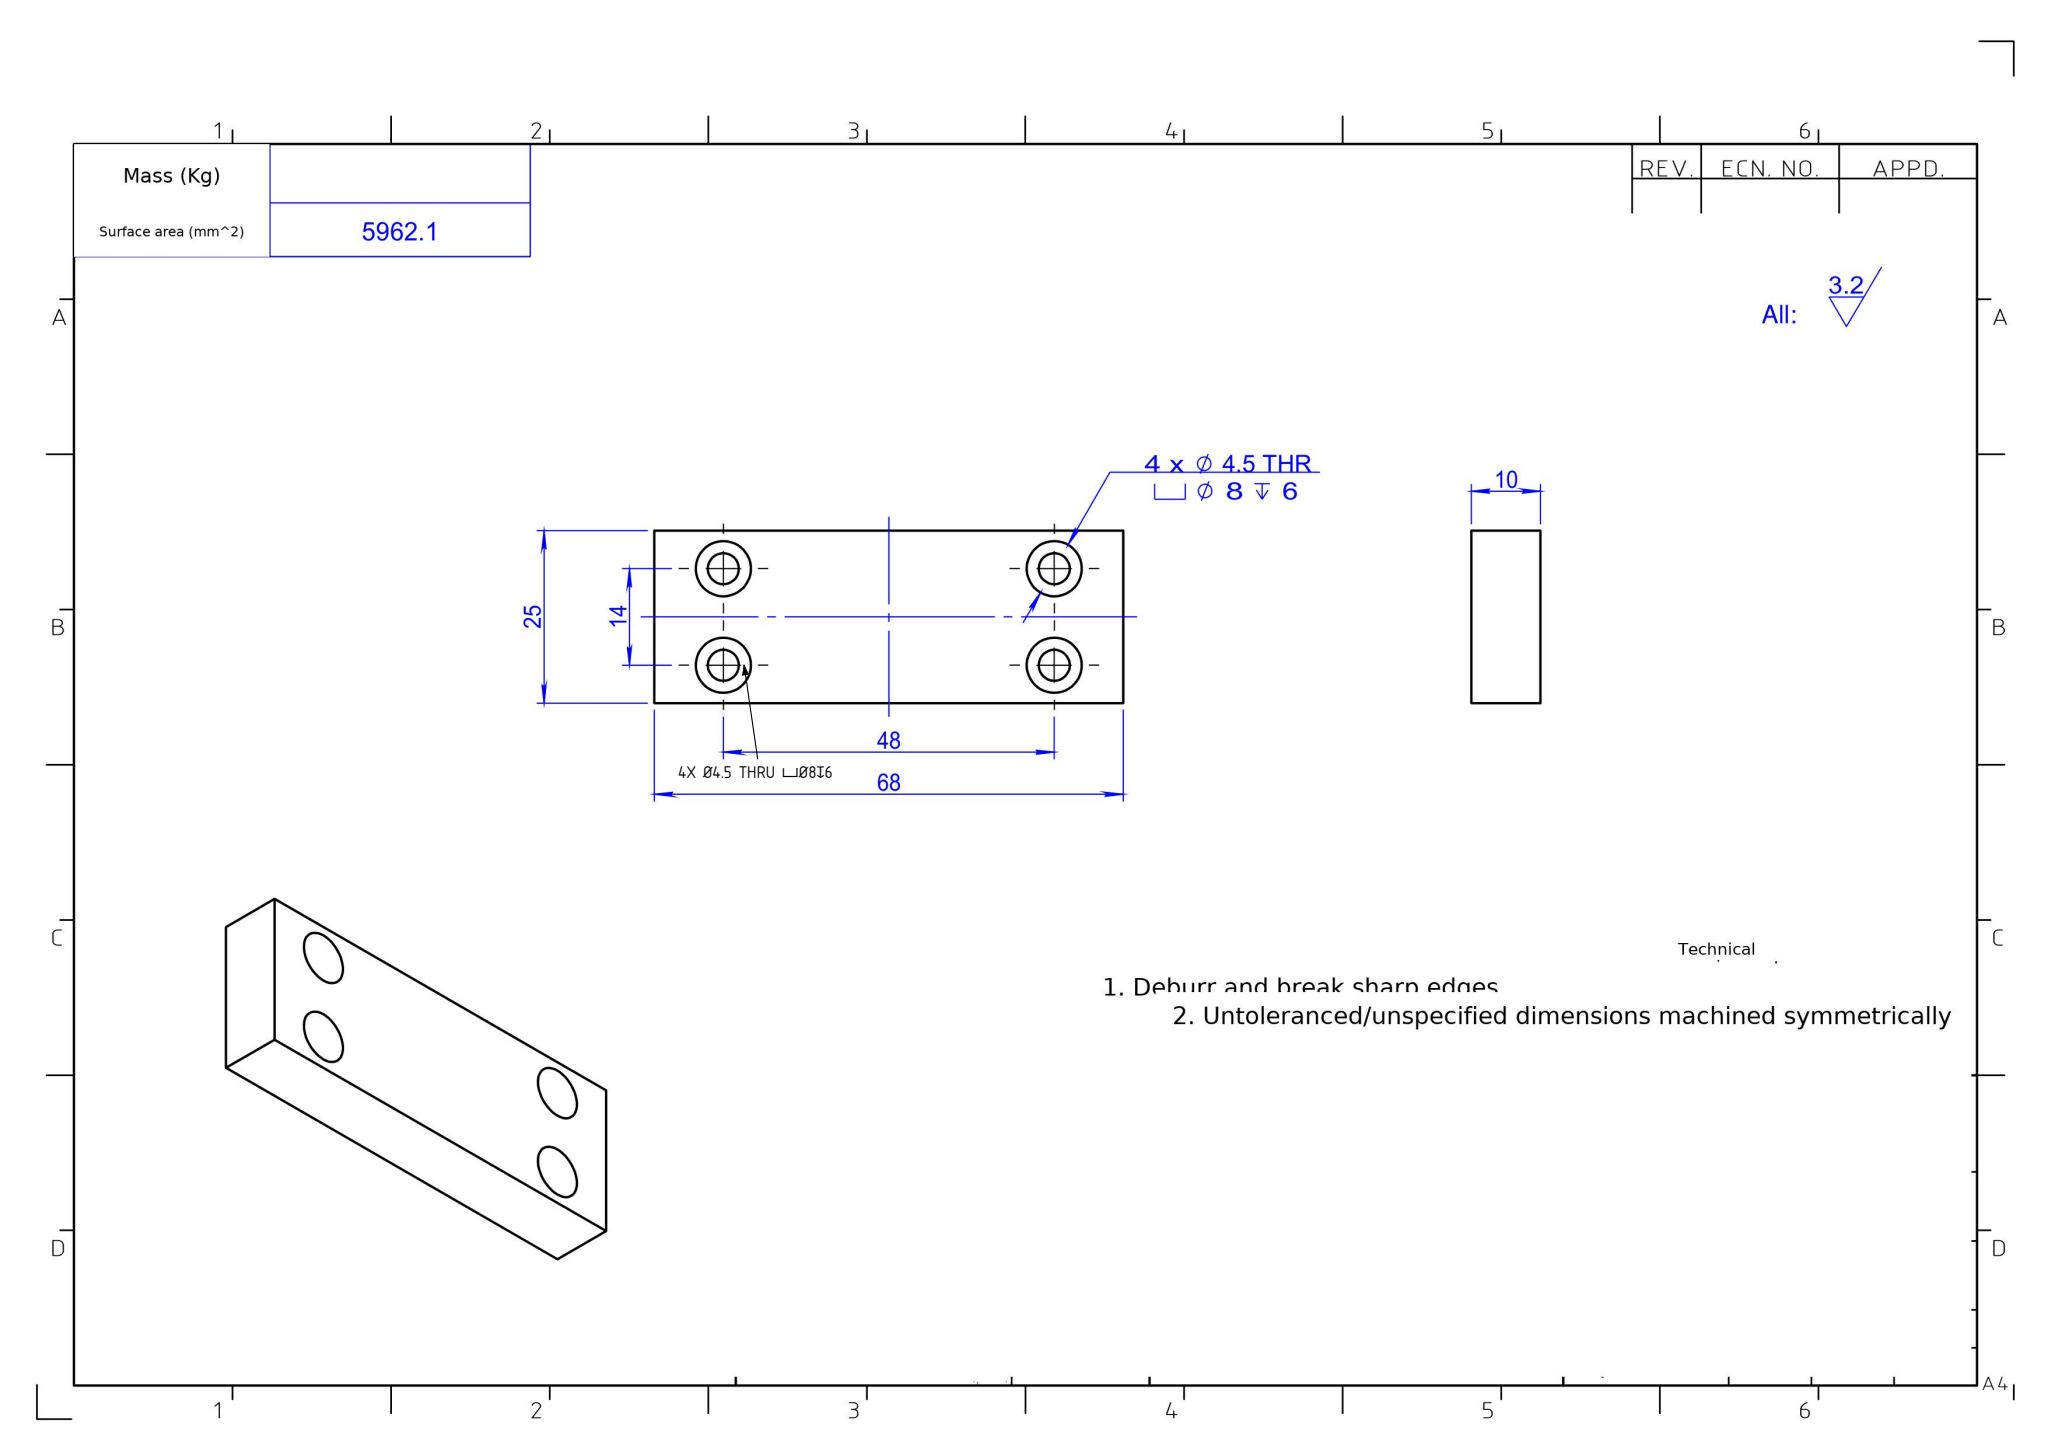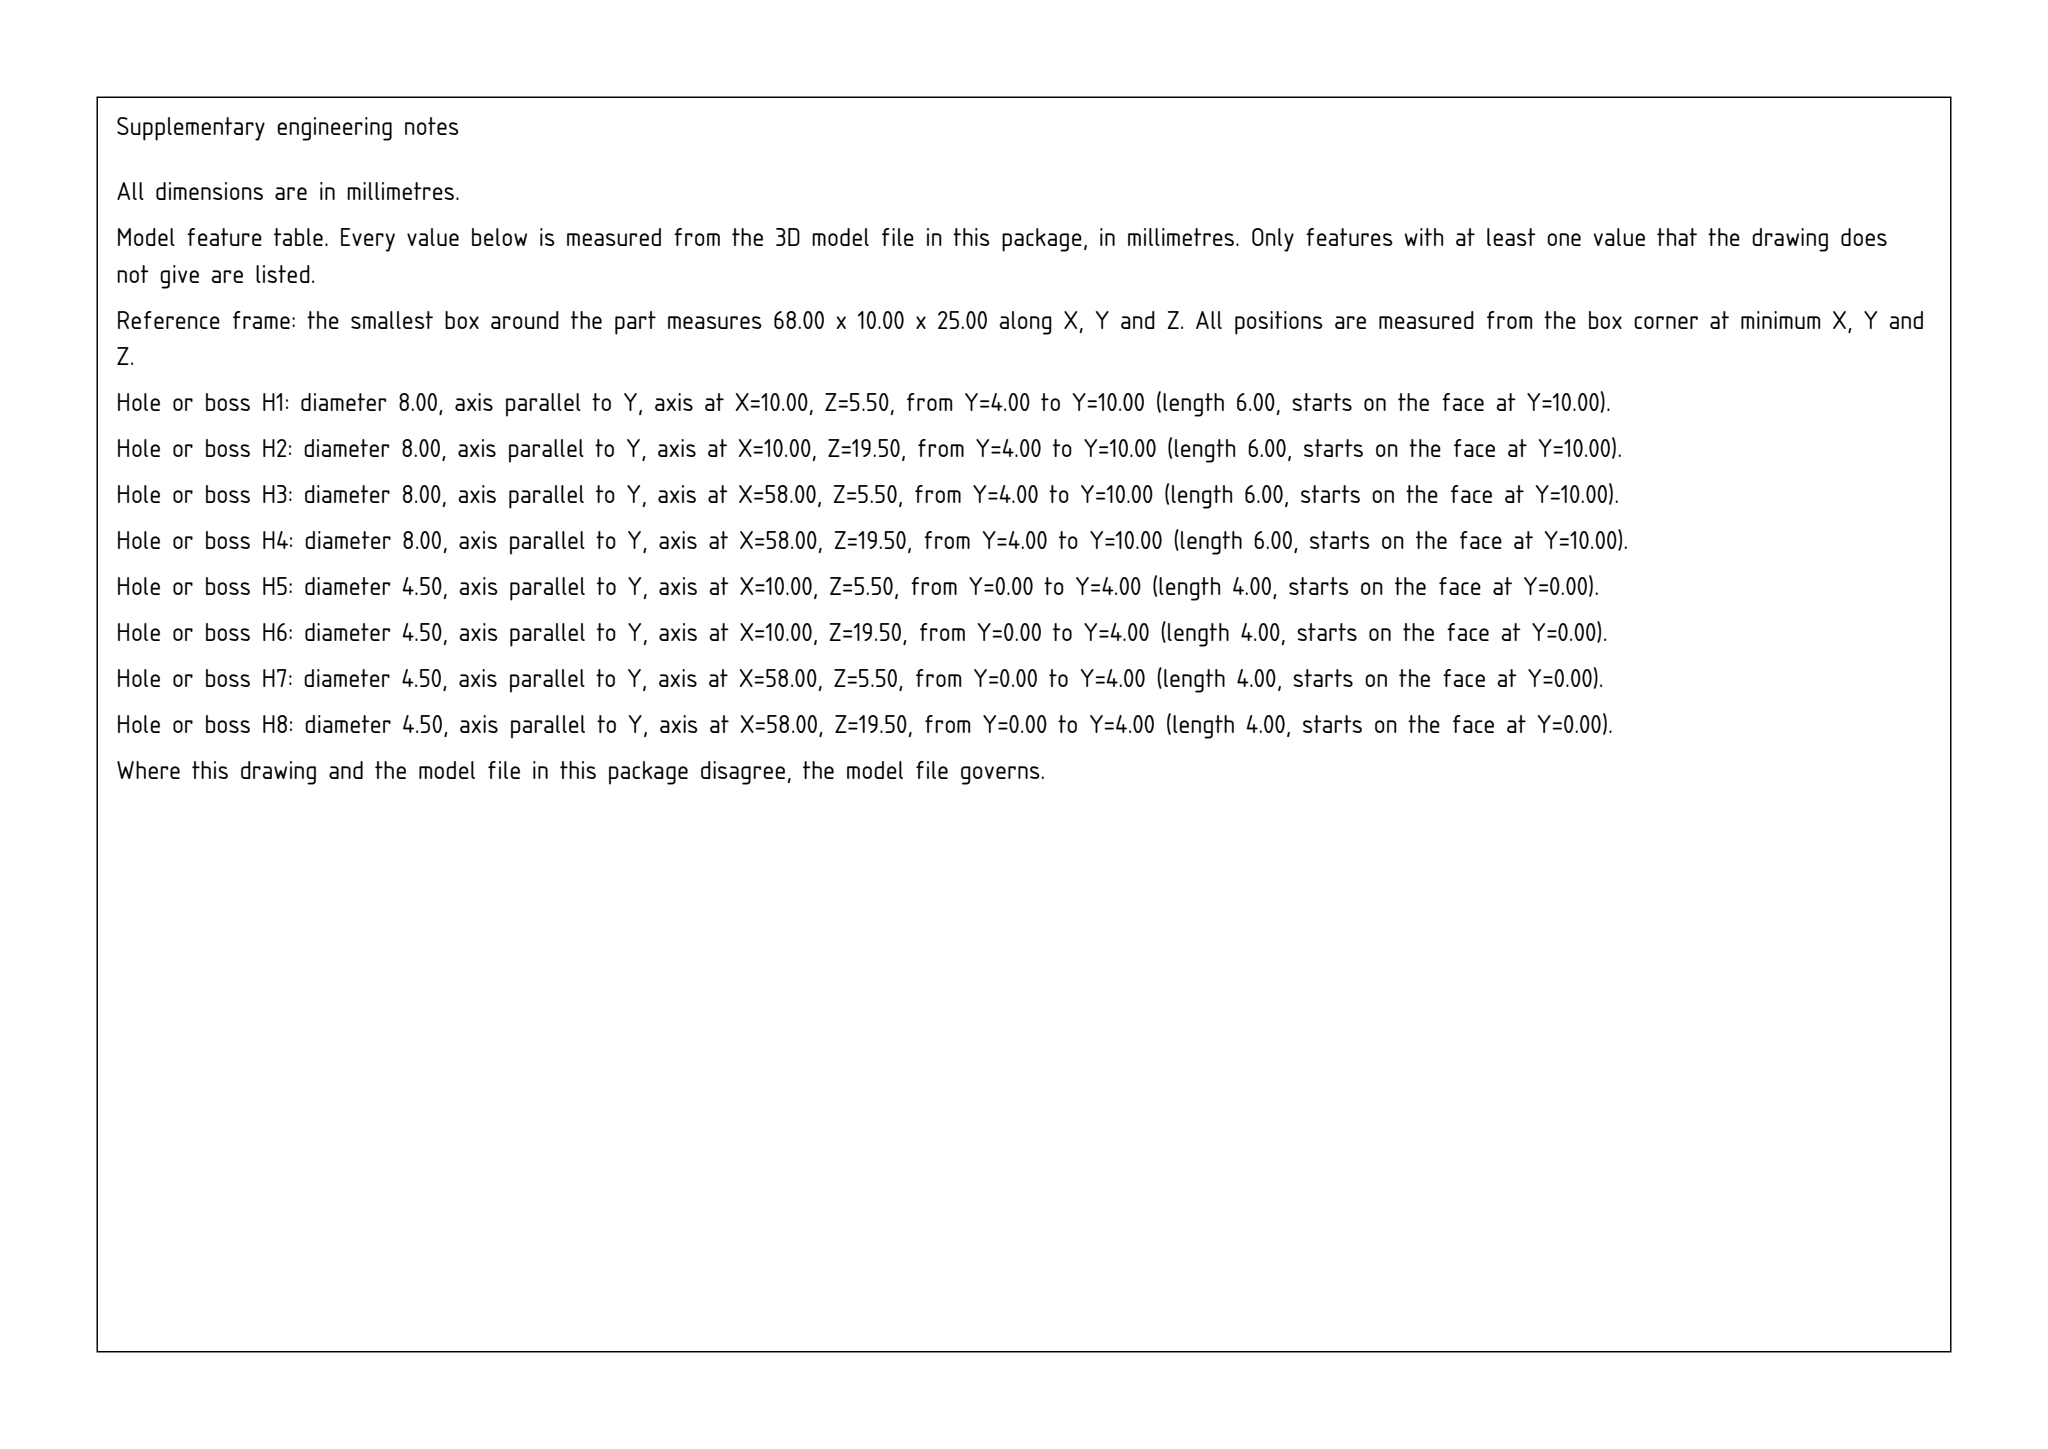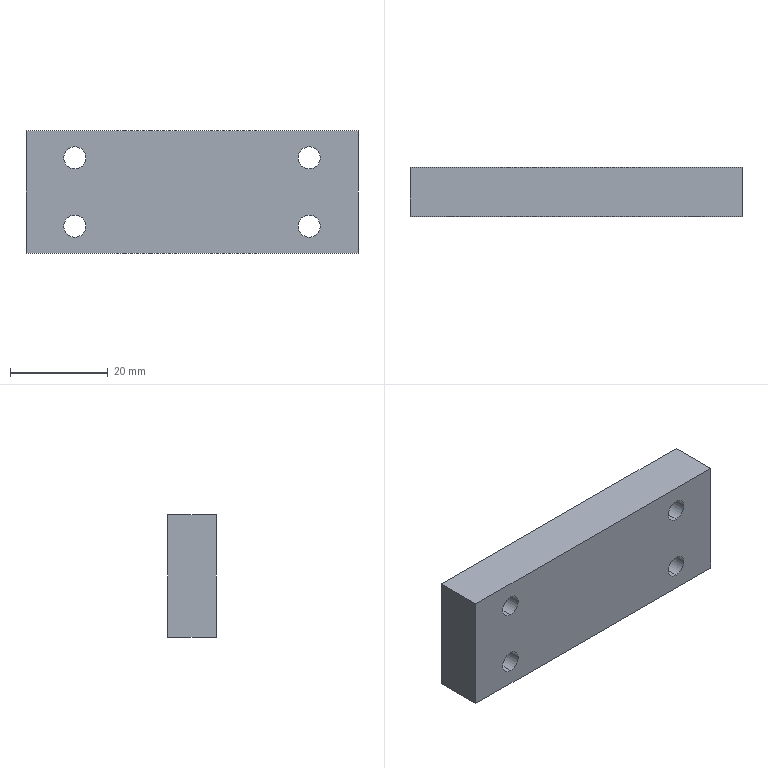Part | SolidWorks | mm | 1 solid | 26 faces | box 68 x 10 x 25 mm | volume 15539 mm3 | cylinder 16 | plane 10 | commonest cylinder face diameters 4.5 x8 8 x8
Drawing notes:
4X Ø4.5 THRU, C'BORE Ø8 DP 6 FROM OPP FACE | from the solid: Ø4.5 bores y=0->4 (4 deep) and Ø8 bores y=4->10 (6 deep) in 10 thk plate; 4+6=10 = full thickness, so Ø4.5 breaks through
build123d program:
from build123d import *

# Parameters (mm, degrees)
SKETCH1_W                                            = 68
SKETCH1_H                                            = 25
EXTRUDE1_DEPTH                                       = 10
COUNTERBORE_FOR_M4_HEX_SOCKET_HEAD_CAP_S_D           = 4.5
COUNTERBORE_FOR_M4_HEX_SOCKET_HEAD_CAP_S_CBORE_D     = 8
COUNTERBORE_FOR_M4_HEX_SOCKET_HEAD_CAP_S_CBORE_DEPTH = 6


with BuildPart() as part:
    # Sketch1 → Extrude1 (new body)
    with BuildSketch(Plane(origin=(0, 0, 0), x_dir=(1, 0, 0), z_dir=(0, 1, 0))):
        Rectangle(SKETCH1_W, SKETCH1_H)
    extrude(amount=EXTRUDE1_DEPTH)

    # Counterbore for M4 Hex Socket Head Cap S (through all)
    with Locations(Plane(origin=(0, 10, 0), x_dir=(-1, 0, 0), z_dir=(0, 1, 0))):
        with Locations((24, 7), (-24, 7), (-24, -7), (24, -7)):
            CounterBoreHole(COUNTERBORE_FOR_M4_HEX_SOCKET_HEAD_CAP_S_D / 2, COUNTERBORE_FOR_M4_HEX_SOCKET_HEAD_CAP_S_CBORE_D / 2, COUNTERBORE_FOR_M4_HEX_SOCKET_HEAD_CAP_S_CBORE_DEPTH)


solid = part.part
STEP:
#1=CARTESIAN_POINT('',(-24.,0.,4.75));
#2=VERTEX_POINT('',#1);
#3=CARTESIAN_POINT('',(-24.,0.,9.25));
#4=VERTEX_POINT('',#3);
#5=CARTESIAN_POINT('',(-24.,0.,7.));
#6=DIRECTION('',(0.,1.,0.));
#7=DIRECTION('',(0.,0.,1.));
#8=AXIS2_PLACEMENT_3D('',#5,#6,#7);
#9=CIRCLE('',#8,2.25);
#10=EDGE_CURVE('',#2,#4,#9,.T.);
#11=ORIENTED_EDGE('',*,*,#10,.F.);
#12=CARTESIAN_POINT('',(-24.,4.,4.75));
#13=VERTEX_POINT('',#12);
#14=CARTESIAN_POINT('',(-24.,10.,4.75));
#15=DIRECTION('',(0.,1.,0.));
#16=VECTOR('',#15,1000.);
#17=LINE('',#14,#16);
#18=EDGE_CURVE('',#2,#13,#17,.T.);
#19=ORIENTED_EDGE('',*,*,#18,.T.);
#20=CARTESIAN_POINT('',(-24.,4.,9.25));
#21=VERTEX_POINT('',#20);
#22=CARTESIAN_POINT('',(-24.,4.,7.));
#23=DIRECTION('',(0.,1.,0.));
#24=DIRECTION('',(0.,0.,1.));
#25=AXIS2_PLACEMENT_3D('',#22,#23,#24);
#26=CIRCLE('',#25,2.25);
#27=EDGE_CURVE('',#13,#21,#26,.T.);
#28=ORIENTED_EDGE('',*,*,#27,.T.);
#29=CARTESIAN_POINT('',(-24.,10.,9.25));
#30=DIRECTION('',(0.,1.,0.));
#31=VECTOR('',#30,1000.);
#32=LINE('',#29,#31);
#33=EDGE_CURVE('',#4,#21,#32,.T.);
#34=ORIENTED_EDGE('',*,*,#33,.F.);
#35=EDGE_LOOP('',(#11,#19,#28,#34));
#36=FACE_OUTER_BOUND('',#35,.T.);
#37=CARTESIAN_POINT('',(-24.,10.,7.));
#38=DIRECTION('',(0.,1.,0.));
#39=DIRECTION('',(0.,0.,1.));
#40=AXIS2_PLACEMENT_3D('',#37,#38,#39);
#41=CYLINDRICAL_SURFACE('',#40,2.25);
#42=ADVANCED_FACE('',(#36),#41,.F.);
#43=CARTESIAN_POINT('',(-24.,4.,3.));
#44=VERTEX_POINT('',#43);
#45=CARTESIAN_POINT('',(-24.,4.,11.));
#46=VERTEX_POINT('',#45);
#47=CARTESIAN_POINT('',(-24.,4.,7.));
#48=DIRECTION('',(0.,1.,0.));
#49=DIRECTION('',(0.,0.,1.));
#50=AXIS2_PLACEMENT_3D('',#47,#48,#49);
#51=CIRCLE('',#50,4.);
#52=EDGE_CURVE('',#44,#46,#51,.T.);
#53=ORIENTED_EDGE('',*,*,#52,.F.);
#54=CARTESIAN_POINT('',(-24.,10.,3.));
#55=VERTEX_POINT('',#54);
#56=CARTESIAN_POINT('',(-24.,10.,3.));
#57=DIRECTION('',(0.,1.,0.));
#58=VECTOR('',#57,1000.);
#59=LINE('',#56,#58);
#60=EDGE_CURVE('',#44,#55,#59,.T.);
#61=ORIENTED_EDGE('',*,*,#60,.T.);
#62=CARTESIAN_POINT('',(-24.,10.,11.));
#63=VERTEX_POINT('',#62);
#64=CARTESIAN_POINT('',(-24.,10.,7.));
#65=DIRECTION('',(0.,1.,0.));
#66=DIRECTION('',(0.,0.,1.));
#67=AXIS2_PLACEMENT_3D('',#64,#65,#66);
#68=CIRCLE('',#67,4.);
#69=EDGE_CURVE('',#55,#63,#68,.T.);
#70=ORIENTED_EDGE('',*,*,#69,.T.);
#71=CARTESIAN_POINT('',(-24.,10.,11.));
#72=DIRECTION('',(0.,1.,0.));
#73=VECTOR('',#72,1000.);
#74=LINE('',#71,#73);
#75=EDGE_CURVE('',#46,#63,#74,.T.);
#76=ORIENTED_EDGE('',*,*,#75,.F.);
#77=EDGE_LOOP('',(#53,#61,#70,#76));
#78=FACE_OUTER_BOUND('',#77,.T.);
#79=CARTESIAN_POINT('',(-24.,10.,7.));
#80=DIRECTION('',(0.,1.,0.));
#81=DIRECTION('',(0.,0.,1.));
#82=AXIS2_PLACEMENT_3D('',#79,#80,#81);
#83=CYLINDRICAL_SURFACE('',#82,4.);
#84=ADVANCED_FACE('',(#78),#83,.F.);
#85=CARTESIAN_POINT('',(24.,0.,4.75));
#86=VERTEX_POINT('',#85);
#87=CARTESIAN_POINT('',(24.,0.,9.25));
#88=VERTEX_POINT('',#87);
#89=CARTESIAN_POINT('',(24.,0.,7.));
#90=DIRECTION('',(0.,1.,0.));
#91=DIRECTION('',(0.,0.,1.));
#92=AXIS2_PLACEMENT_3D('',#89,#90,#91);
#93=CIRCLE('',#92,2.25);
#94=EDGE_CURVE('',#86,#88,#93,.T.);
#95=ORIENTED_EDGE('',*,*,#94,.F.);
#96=CARTESIAN_POINT('',(24.,4.,4.75));
#97=VERTEX_POINT('',#96);
#98=CARTESIAN_POINT('',(24.,10.,4.75));
#99=DIRECTION('',(0.,1.,0.));
#100=VECTOR('',#99,1000.);
#101=LINE('',#98,#100);
#102=EDGE_CURVE('',#86,#97,#101,.T.);
#103=ORIENTED_EDGE('',*,*,#102,.T.);
#104=CARTESIAN_POINT('',(24.,4.,9.25));
#105=VERTEX_POINT('',#104);
#106=CARTESIAN_POINT('',(24.,4.,7.));
#107=DIRECTION('',(0.,1.,0.));
#108=DIRECTION('',(0.,0.,1.));
#109=AXIS2_PLACEMENT_3D('',#106,#107,#108);
#110=CIRCLE('',#109,2.25);
#111=EDGE_CURVE('',#97,#105,#110,.T.);
#112=ORIENTED_EDGE('',*,*,#111,.T.);
#113=CARTESIAN_POINT('',(24.,10.,9.25));
#114=DIRECTION('',(0.,1.,0.));
#115=VECTOR('',#114,1000.);
#116=LINE('',#113,#115);
#117=EDGE_CURVE('',#88,#105,#116,.T.);
#118=ORIENTED_EDGE('',*,*,#117,.F.);
#119=EDGE_LOOP('',(#95,#103,#112,#118));
#120=FACE_OUTER_BOUND('',#119,.T.);
#121=CARTESIAN_POINT('',(24.,10.,7.));
#122=DIRECTION('',(0.,1.,0.));
#123=DIRECTION('',(0.,0.,1.));
#124=AXIS2_PLACEMENT_3D('',#121,#122,#123);
#125=CYLINDRICAL_SURFACE('',#124,2.25);
#126=ADVANCED_FACE('',(#120),#125,.F.);
#127=CARTESIAN_POINT('',(24.,4.,3.));
#128=VERTEX_POINT('',#127);
#129=CARTESIAN_POINT('',(24.,4.,11.));
#130=VERTEX_POINT('',#129);
#131=CARTESIAN_POINT('',(24.,4.,7.));
#132=DIRECTION('',(0.,1.,0.));
#133=DIRECTION('',(0.,0.,1.));
#134=AXIS2_PLACEMENT_3D('',#131,#132,#133);
#135=CIRCLE('',#134,4.);
#136=EDGE_CURVE('',#128,#130,#135,.T.);
#137=ORIENTED_EDGE('',*,*,#136,.F.);
#138=CARTESIAN_POINT('',(24.,10.,3.));
#139=VERTEX_POINT('',#138);
#140=CARTESIAN_POINT('',(24.,10.,3.));
#141=DIRECTION('',(0.,1.,0.));
#142=VECTOR('',#141,1000.);
#143=LINE('',#140,#142);
#144=EDGE_CURVE('',#128,#139,#143,.T.);
#145=ORIENTED_EDGE('',*,*,#144,.T.);
#146=CARTESIAN_POINT('',(24.,10.,11.));
#147=VERTEX_POINT('',#146);
#148=CARTESIAN_POINT('',(24.,10.,7.));
#149=DIRECTION('',(0.,1.,0.));
#150=DIRECTION('',(0.,0.,1.));
#151=AXIS2_PLACEMENT_3D('',#148,#149,#150);
#152=CIRCLE('',#151,4.);
#153=EDGE_CURVE('',#139,#147,#152,.T.);
#154=ORIENTED_EDGE('',*,*,#153,.T.);
#155=CARTESIAN_POINT('',(24.,10.,11.));
#156=DIRECTION('',(0.,1.,0.));
#157=VECTOR('',#156,1000.);
#158=LINE('',#155,#157);
#159=EDGE_CURVE('',#130,#147,#158,.T.);
#160=ORIENTED_EDGE('',*,*,#159,.F.);
#161=EDGE_LOOP('',(#137,#145,#154,#160));
#162=FACE_OUTER_BOUND('',#161,.T.);
#163=CARTESIAN_POINT('',(24.,10.,7.));
#164=DIRECTION('',(0.,1.,0.));
#165=DIRECTION('',(0.,0.,1.));
#166=AXIS2_PLACEMENT_3D('',#163,#164,#165);
#167=CYLINDRICAL_SURFACE('',#166,4.);
#168=ADVANCED_FACE('',(#162),#167,.F.);
#169=CARTESIAN_POINT('',(24.,0.,-9.25));
#170=VERTEX_POINT('',#169);
#171=CARTESIAN_POINT('',(24.,0.,-4.75));
#172=VERTEX_POINT('',#171);
#173=CARTESIAN_POINT('',(24.,0.,-7.));
#174=DIRECTION('',(0.,1.,0.));
#175=DIRECTION('',(0.,0.,1.));
#176=AXIS2_PLACEMENT_3D('',#173,#174,#175);
#177=CIRCLE('',#176,2.25);
#178=EDGE_CURVE('',#170,#172,#177,.T.);
#179=ORIENTED_EDGE('',*,*,#178,.F.);
#180=CARTESIAN_POINT('',(24.,4.,-9.25));
#181=VERTEX_POINT('',#180);
#182=CARTESIAN_POINT('',(24.,10.,-9.25));
#183=DIRECTION('',(0.,1.,0.));
#184=VECTOR('',#183,1000.);
#185=LINE('',#182,#184);
#186=EDGE_CURVE('',#170,#181,#185,.T.);
#187=ORIENTED_EDGE('',*,*,#186,.T.);
#188=CARTESIAN_POINT('',(24.,4.,-4.75));
#189=VERTEX_POINT('',#188);
#190=CARTESIAN_POINT('',(24.,4.,-7.));
#191=DIRECTION('',(0.,1.,0.));
#192=DIRECTION('',(0.,0.,1.));
#193=AXIS2_PLACEMENT_3D('',#190,#191,#192);
#194=CIRCLE('',#193,2.25);
#195=EDGE_CURVE('',#181,#189,#194,.T.);
#196=ORIENTED_EDGE('',*,*,#195,.T.);
#197=CARTESIAN_POINT('',(24.,10.,-4.75));
#198=DIRECTION('',(0.,1.,0.));
#199=VECTOR('',#198,1000.);
#200=LINE('',#197,#199);
#201=EDGE_CURVE('',#172,#189,#200,.T.);
#202=ORIENTED_EDGE('',*,*,#201,.F.);
#203=EDGE_LOOP('',(#179,#187,#196,#202));
#204=FACE_OUTER_BOUND('',#203,.T.);
#205=CARTESIAN_POINT('',(24.,10.,-7.));
#206=DIRECTION('',(0.,1.,0.));
#207=DIRECTION('',(0.,0.,1.));
#208=AXIS2_PLACEMENT_3D('',#205,#206,#207);
#209=CYLINDRICAL_SURFACE('',#208,2.25);
#210=ADVANCED_FACE('',(#204),#209,.F.);
#211=CARTESIAN_POINT('',(24.,4.,-11.));
#212=VERTEX_POINT('',#211);
#213=CARTESIAN_POINT('',(24.,4.,-3.));
#214=VERTEX_POINT('',#213);
#215=CARTESIAN_POINT('',(24.,4.,-7.));
#216=DIRECTION('',(0.,1.,0.));
#217=DIRECTION('',(0.,0.,1.));
#218=AXIS2_PLACEMENT_3D('',#215,#216,#217);
#219=CIRCLE('',#218,4.);
#220=EDGE_CURVE('',#212,#214,#219,.T.);
#221=ORIENTED_EDGE('',*,*,#220,.F.);
#222=CARTESIAN_POINT('',(24.,10.,-11.));
#223=VERTEX_POINT('',#222);
#224=CARTESIAN_POINT('',(24.,10.,-11.));
#225=DIRECTION('',(0.,1.,0.));
#226=VECTOR('',#225,1000.);
#227=LINE('',#224,#226);
#228=EDGE_CURVE('',#212,#223,#227,.T.);
#229=ORIENTED_EDGE('',*,*,#228,.T.);
#230=CARTESIAN_POINT('',(24.,10.,-3.));
#231=VERTEX_POINT('',#230);
#232=CARTESIAN_POINT('',(24.,10.,-7.));
#233=DIRECTION('',(0.,1.,0.));
#234=DIRECTION('',(0.,0.,1.));
#235=AXIS2_PLACEMENT_3D('',#232,#233,#234);
#236=CIRCLE('',#235,4.);
#237=EDGE_CURVE('',#223,#231,#236,.T.);
#238=ORIENTED_EDGE('',*,*,#237,.T.);
#239=CARTESIAN_POINT('',(24.,10.,-3.));
#240=DIRECTION('',(0.,1.,0.));
#241=VECTOR('',#240,1000.);
#242=LINE('',#239,#241);
#243=EDGE_CURVE('',#214,#231,#242,.T.);
#244=ORIENTED_EDGE('',*,*,#243,.F.);
#245=EDGE_LOOP('',(#221,#229,#238,#244));
#246=FACE_OUTER_BOUND('',#245,.T.);
#247=CARTESIAN_POINT('',(24.,10.,-7.));
#248=DIRECTION('',(0.,1.,0.));
#249=DIRECTION('',(0.,0.,1.));
#250=AXIS2_PLACEMENT_3D('',#247,#248,#249);
#251=CYLINDRICAL_SURFACE('',#250,4.);
#252=ADVANCED_FACE('',(#246),#251,.F.);
#253=CARTESIAN_POINT('',(-24.,0.,-9.25));
#254=VERTEX_POINT('',#253);
#255=CARTESIAN_POINT('',(-24.,0.,-4.75));
#256=VERTEX_POINT('',#255);
#257=CARTESIAN_POINT('',(-24.,0.,-7.));
#258=DIRECTION('',(0.,1.,0.));
#259=DIRECTION('',(0.,0.,1.));
#260=AXIS2_PLACEMENT_3D('',#257,#258,#259);
#261=CIRCLE('',#260,2.25);
#262=EDGE_CURVE('',#254,#256,#261,.T.);
#263=ORIENTED_EDGE('',*,*,#262,.F.);
#264=CARTESIAN_POINT('',(-24.,4.,-9.25));
#265=VERTEX_POINT('',#264);
#266=CARTESIAN_POINT('',(-24.,10.,-9.25));
#267=DIRECTION('',(0.,1.,0.));
#268=VECTOR('',#267,1000.);
#269=LINE('',#266,#268);
#270=EDGE_CURVE('',#254,#265,#269,.T.);
#271=ORIENTED_EDGE('',*,*,#270,.T.);
#272=CARTESIAN_POINT('',(-24.,4.,-4.75));
#273=VERTEX_POINT('',#272);
#274=CARTESIAN_POINT('',(-24.,4.,-7.));
#275=DIRECTION('',(0.,1.,0.));
#276=DIRECTION('',(0.,0.,1.));
#277=AXIS2_PLACEMENT_3D('',#274,#275,#276);
#278=CIRCLE('',#277,2.25);
#279=EDGE_CURVE('',#265,#273,#278,.T.);
#280=ORIENTED_EDGE('',*,*,#279,.T.);
#281=CARTESIAN_POINT('',(-24.,10.,-4.75));
#282=DIRECTION('',(0.,1.,0.));
#283=VECTOR('',#282,1000.);
#284=LINE('',#281,#283);
#285=EDGE_CURVE('',#256,#273,#284,.T.);
#286=ORIENTED_EDGE('',*,*,#285,.F.);
#287=EDGE_LOOP('',(#263,#271,#280,#286));
#288=FACE_OUTER_BOUND('',#287,.T.);
#289=CARTESIAN_POINT('',(-24.,10.,-7.));
#290=DIRECTION('',(0.,1.,0.));
#291=DIRECTION('',(0.,0.,1.));
#292=AXIS2_PLACEMENT_3D('',#289,#290,#291);
#293=CYLINDRICAL_SURFACE('',#292,2.25);
#294=ADVANCED_FACE('',(#288),#293,.F.);
#295=CARTESIAN_POINT('',(-24.,4.,-11.));
#296=VERTEX_POINT('',#295);
#297=CARTESIAN_POINT('',(-24.,4.,-3.));
#298=VERTEX_POINT('',#297);
#299=CARTESIAN_POINT('',(-24.,4.,-7.));
#300=DIRECTION('',(0.,1.,0.));
#301=DIRECTION('',(0.,0.,1.));
#302=AXIS2_PLACEMENT_3D('',#299,#300,#301);
#303=CIRCLE('',#302,4.);
#304=EDGE_CURVE('',#296,#298,#303,.T.);
#305=ORIENTED_EDGE('',*,*,#304,.F.);
#306=CARTESIAN_POINT('',(-24.,10.,-11.));
#307=VERTEX_POINT('',#306);
#308=CARTESIAN_POINT('',(-24.,10.,-11.));
#309=DIRECTION('',(0.,1.,0.));
#310=VECTOR('',#309,1000.);
#311=LINE('',#308,#310);
#312=EDGE_CURVE('',#296,#307,#311,.T.);
#313=ORIENTED_EDGE('',*,*,#312,.T.);
#314=CARTESIAN_POINT('',(-24.,10.,-3.));
#315=VERTEX_POINT('',#314);
#316=CARTESIAN_POINT('',(-24.,10.,-7.));
#317=DIRECTION('',(0.,1.,0.));
#318=DIRECTION('',(0.,0.,1.));
#319=AXIS2_PLACEMENT_3D('',#316,#317,#318);
#320=CIRCLE('',#319,4.);
#321=EDGE_CURVE('',#307,#315,#320,.T.);
#322=ORIENTED_EDGE('',*,*,#321,.T.);
#323=CARTESIAN_POINT('',(-24.,10.,-3.));
#324=DIRECTION('',(0.,1.,0.));
#325=VECTOR('',#324,1000.);
#326=LINE('',#323,#325);
#327=EDGE_CURVE('',#298,#315,#326,.T.);
#328=ORIENTED_EDGE('',*,*,#327,.F.);
#329=EDGE_LOOP('',(#305,#313,#322,#328));
#330=FACE_OUTER_BOUND('',#329,.T.);
#331=CARTESIAN_POINT('',(-24.,10.,-7.));
#332=DIRECTION('',(0.,1.,0.));
#333=DIRECTION('',(0.,0.,1.));
#334=AXIS2_PLACEMENT_3D('',#331,#332,#333);
#335=CYLINDRICAL_SURFACE('',#334,4.);
#336=ADVANCED_FACE('',(#330),#335,.F.);
#337=CARTESIAN_POINT('',(-34.,0.,-12.5));
#338=VERTEX_POINT('',#337);
#339=CARTESIAN_POINT('',(-34.,0.,12.5));
#340=VERTEX_POINT('',#339);
#341=CARTESIAN_POINT('',(-34.,0.,-12.5));
#342=DIRECTION('',(0.,0.,1.));
#343=VECTOR('',#342,1000.);
#344=LINE('',#341,#343);
#345=EDGE_CURVE('',#338,#340,#344,.T.);
#346=ORIENTED_EDGE('',*,*,#345,.T.);
#347=CARTESIAN_POINT('',(-34.,10.,12.5));
#348=VERTEX_POINT('',#347);
#349=CARTESIAN_POINT('',(-34.,10.,12.5));
#350=DIRECTION('',(0.,-1.,0.));
#351=VECTOR('',#350,1000.);
#352=LINE('',#349,#351);
#353=EDGE_CURVE('',#348,#340,#352,.T.);
#354=ORIENTED_EDGE('',*,*,#353,.F.);
#355=CARTESIAN_POINT('',(-34.,10.,-12.5));
#356=VERTEX_POINT('',#355);
#357=CARTESIAN_POINT('',(-34.,10.,-12.5));
#358=DIRECTION('',(0.,0.,1.));
#359=VECTOR('',#358,1000.);
#360=LINE('',#357,#359);
#361=EDGE_CURVE('',#356,#348,#360,.T.);
#362=ORIENTED_EDGE('',*,*,#361,.F.);
#363=CARTESIAN_POINT('',(-34.,10.,-12.5));
#364=DIRECTION('',(0.,-1.,0.));
#365=VECTOR('',#364,1000.);
#366=LINE('',#363,#365);
#367=EDGE_CURVE('',#356,#338,#366,.T.);
#368=ORIENTED_EDGE('',*,*,#367,.T.);
#369=EDGE_LOOP('',(#346,#354,#362,#368));
#370=FACE_OUTER_BOUND('',#369,.T.);
#371=CARTESIAN_POINT('',(-34.,10.,-12.5));
#372=DIRECTION('',(1.,0.,0.));
#373=DIRECTION('',(0.,0.,-1.));
#374=AXIS2_PLACEMENT_3D('',#371,#372,#373);
#375=PLANE('',#374);
#376=ADVANCED_FACE('',(#370),#375,.F.);
#377=CARTESIAN_POINT('',(34.,0.,12.5));
#378=VERTEX_POINT('',#377);
#379=CARTESIAN_POINT('',(-34.,0.,12.5));
#380=DIRECTION('',(1.,0.,0.));
#381=VECTOR('',#380,1000.);
#382=LINE('',#379,#381);
#383=EDGE_CURVE('',#340,#378,#382,.T.);
#384=ORIENTED_EDGE('',*,*,#383,.T.);
#385=CARTESIAN_POINT('',(34.,10.,12.5));
#386=VERTEX_POINT('',#385);
#387=CARTESIAN_POINT('',(34.,10.,12.5));
#388=DIRECTION('',(0.,-1.,0.));
#389=VECTOR('',#388,1000.);
#390=LINE('',#387,#389);
#391=EDGE_CURVE('',#386,#378,#390,.T.);
#392=ORIENTED_EDGE('',*,*,#391,.F.);
#393=CARTESIAN_POINT('',(-34.,10.,12.5));
#394=DIRECTION('',(1.,0.,0.));
#395=VECTOR('',#394,1000.);
#396=LINE('',#393,#395);
#397=EDGE_CURVE('',#348,#386,#396,.T.);
#398=ORIENTED_EDGE('',*,*,#397,.F.);
#399=ORIENTED_EDGE('',*,*,#353,.T.);
#400=EDGE_LOOP('',(#384,#392,#398,#399));
#401=FACE_OUTER_BOUND('',#400,.T.);
#402=CARTESIAN_POINT('',(-34.,10.,12.5));
#403=DIRECTION('',(0.,0.,-1.));
#404=DIRECTION('',(-1.,0.,0.));
#405=AXIS2_PLACEMENT_3D('',#402,#403,#404);
#406=PLANE('',#405);
#407=ADVANCED_FACE('',(#401),#406,.F.);
#408=CARTESIAN_POINT('',(34.,0.,-12.5));
#409=VERTEX_POINT('',#408);
#410=CARTESIAN_POINT('',(34.,0.,-12.5));
#411=DIRECTION('',(0.,0.,-1.));
#412=VECTOR('',#411,1000.);
#413=LINE('',#410,#412);
#414=EDGE_CURVE('',#378,#409,#413,.T.);
#415=ORIENTED_EDGE('',*,*,#414,.T.);
#416=CARTESIAN_POINT('',(34.,10.,-12.5));
#417=VERTEX_POINT('',#416);
#418=CARTESIAN_POINT('',(34.,10.,-12.5));
#419=DIRECTION('',(0.,-1.,0.));
#420=VECTOR('',#419,1000.);
#421=LINE('',#418,#420);
#422=EDGE_CURVE('',#417,#409,#421,.T.);
#423=ORIENTED_EDGE('',*,*,#422,.F.);
#424=CARTESIAN_POINT('',(34.,10.,-12.5));
#425=DIRECTION('',(0.,0.,-1.));
#426=VECTOR('',#425,1000.);
#427=LINE('',#424,#426);
#428=EDGE_CURVE('',#386,#417,#427,.T.);
#429=ORIENTED_EDGE('',*,*,#428,.F.);
#430=ORIENTED_EDGE('',*,*,#391,.T.);
#431=EDGE_LOOP('',(#415,#423,#429,#430));
#432=FACE_OUTER_BOUND('',#431,.T.);
#433=CARTESIAN_POINT('',(34.,10.,-12.5));
#434=DIRECTION('',(-1.,0.,0.));
#435=DIRECTION('',(0.,0.,1.));
#436=AXIS2_PLACEMENT_3D('',#433,#434,#435);
#437=PLANE('',#436);
#438=ADVANCED_FACE('',(#432),#437,.F.);
#439=CARTESIAN_POINT('',(-34.,0.,-12.5));
#440=DIRECTION('',(-1.,0.,0.));
#441=VECTOR('',#440,1000.);
#442=LINE('',#439,#441);
#443=EDGE_CURVE('',#409,#338,#442,.T.);
#444=ORIENTED_EDGE('',*,*,#443,.T.);
#445=ORIENTED_EDGE('',*,*,#367,.F.);
#446=CARTESIAN_POINT('',(-34.,10.,-12.5));
#447=DIRECTION('',(-1.,0.,0.));
#448=VECTOR('',#447,1000.);
#449=LINE('',#446,#448);
#450=EDGE_CURVE('',#417,#356,#449,.T.);
#451=ORIENTED_EDGE('',*,*,#450,.F.);
#452=ORIENTED_EDGE('',*,*,#422,.T.);
#453=EDGE_LOOP('',(#444,#445,#451,#452));
#454=FACE_OUTER_BOUND('',#453,.T.);
#455=CARTESIAN_POINT('',(-34.,10.,-12.5));
#456=DIRECTION('',(0.,0.,1.));
#457=DIRECTION('',(1.,0.,0.));
#458=AXIS2_PLACEMENT_3D('',#455,#456,#457);
#459=PLANE('',#458);
#460=ADVANCED_FACE('',(#454),#459,.F.);
#461=CARTESIAN_POINT('',(-24.,10.,7.));
#462=DIRECTION('',(0.,1.,0.));
#463=DIRECTION('',(0.,0.,1.));
#464=AXIS2_PLACEMENT_3D('',#461,#462,#463);
#465=CIRCLE('',#464,4.);
#466=EDGE_CURVE('',#63,#55,#465,.T.);
#467=ORIENTED_EDGE('',*,*,#466,.F.);
#468=ORIENTED_EDGE('',*,*,#69,.F.);
#469=EDGE_LOOP('',(#467,#468));
#470=FACE_BOUND('',#469,.T.);
#471=CARTESIAN_POINT('',(24.,10.,7.));
#472=DIRECTION('',(0.,1.,0.));
#473=DIRECTION('',(0.,0.,1.));
#474=AXIS2_PLACEMENT_3D('',#471,#472,#473);
#475=CIRCLE('',#474,4.);
#476=EDGE_CURVE('',#147,#139,#475,.T.);
#477=ORIENTED_EDGE('',*,*,#476,.F.);
#478=ORIENTED_EDGE('',*,*,#153,.F.);
#479=EDGE_LOOP('',(#477,#478));
#480=FACE_BOUND('',#479,.T.);
#481=CARTESIAN_POINT('',(24.,10.,-7.));
#482=DIRECTION('',(0.,1.,0.));
#483=DIRECTION('',(0.,0.,1.));
#484=AXIS2_PLACEMENT_3D('',#481,#482,#483);
#485=CIRCLE('',#484,4.);
#486=EDGE_CURVE('',#231,#223,#485,.T.);
#487=ORIENTED_EDGE('',*,*,#486,.F.);
#488=ORIENTED_EDGE('',*,*,#237,.F.);
#489=EDGE_LOOP('',(#487,#488));
#490=FACE_BOUND('',#489,.T.);
#491=CARTESIAN_POINT('',(-24.,10.,-7.));
#492=DIRECTION('',(0.,1.,0.));
#493=DIRECTION('',(0.,0.,1.));
#494=AXIS2_PLACEMENT_3D('',#491,#492,#493);
#495=CIRCLE('',#494,4.);
#496=EDGE_CURVE('',#315,#307,#495,.T.);
#497=ORIENTED_EDGE('',*,*,#496,.F.);
#498=ORIENTED_EDGE('',*,*,#321,.F.);
#499=EDGE_LOOP('',(#497,#498));
#500=FACE_BOUND('',#499,.T.);
#501=ORIENTED_EDGE('',*,*,#361,.T.);
#502=ORIENTED_EDGE('',*,*,#397,.T.);
#503=ORIENTED_EDGE('',*,*,#428,.T.);
#504=ORIENTED_EDGE('',*,*,#450,.T.);
#505=EDGE_LOOP('',(#501,#502,#503,#504));
#506=FACE_OUTER_BOUND('',#505,.T.);
#507=CARTESIAN_POINT('',(-34.,10.,12.5));
#508=DIRECTION('',(0.,1.,0.));
#509=DIRECTION('',(0.,0.,1.));
#510=AXIS2_PLACEMENT_3D('',#507,#508,#509);
#511=PLANE('',#510);
#512=ADVANCED_FACE('',(#470,#480,#490,#500,#506),#511,.T.);
#513=CARTESIAN_POINT('',(-24.,0.,7.));
#514=DIRECTION('',(0.,1.,0.));
#515=DIRECTION('',(0.,0.,1.));
#516=AXIS2_PLACEMENT_3D('',#513,#514,#515);
#517=CIRCLE('',#516,2.25);
#518=EDGE_CURVE('',#4,#2,#517,.T.);
#519=ORIENTED_EDGE('',*,*,#518,.T.);
#520=ORIENTED_EDGE('',*,*,#10,.T.);
#521=EDGE_LOOP('',(#519,#520));
#522=FACE_BOUND('',#521,.T.);
#523=CARTESIAN_POINT('',(24.,0.,7.));
#524=DIRECTION('',(0.,1.,0.));
#525=DIRECTION('',(0.,0.,1.));
#526=AXIS2_PLACEMENT_3D('',#523,#524,#525);
#527=CIRCLE('',#526,2.25);
#528=EDGE_CURVE('',#88,#86,#527,.T.);
#529=ORIENTED_EDGE('',*,*,#528,.T.);
#530=ORIENTED_EDGE('',*,*,#94,.T.);
#531=EDGE_LOOP('',(#529,#530));
#532=FACE_BOUND('',#531,.T.);
#533=CARTESIAN_POINT('',(24.,0.,-7.));
#534=DIRECTION('',(0.,1.,0.));
#535=DIRECTION('',(0.,0.,1.));
#536=AXIS2_PLACEMENT_3D('',#533,#534,#535);
#537=CIRCLE('',#536,2.25);
#538=EDGE_CURVE('',#172,#170,#537,.T.);
#539=ORIENTED_EDGE('',*,*,#538,.T.);
#540=ORIENTED_EDGE('',*,*,#178,.T.);
#541=EDGE_LOOP('',(#539,#540));
#542=FACE_BOUND('',#541,.T.);
#543=CARTESIAN_POINT('',(-24.,0.,-7.));
#544=DIRECTION('',(0.,1.,0.));
#545=DIRECTION('',(0.,0.,1.));
#546=AXIS2_PLACEMENT_3D('',#543,#544,#545);
#547=CIRCLE('',#546,2.25);
#548=EDGE_CURVE('',#256,#254,#547,.T.);
#549=ORIENTED_EDGE('',*,*,#548,.T.);
#550=ORIENTED_EDGE('',*,*,#262,.T.);
#551=EDGE_LOOP('',(#549,#550));
#552=FACE_BOUND('',#551,.T.);
#553=ORIENTED_EDGE('',*,*,#345,.F.);
#554=ORIENTED_EDGE('',*,*,#443,.F.);
#555=ORIENTED_EDGE('',*,*,#414,.F.);
#556=ORIENTED_EDGE('',*,*,#383,.F.);
#557=EDGE_LOOP('',(#553,#554,#555,#556));
#558=FACE_OUTER_BOUND('',#557,.T.);
#559=CARTESIAN_POINT('',(-34.,0.,12.5));
#560=DIRECTION('',(0.,1.,0.));
#561=DIRECTION('',(0.,0.,1.));
#562=AXIS2_PLACEMENT_3D('',#559,#560,#561);
#563=PLANE('',#562);
#564=ADVANCED_FACE('',(#522,#532,#542,#552,#558),#563,.F.);
#565=ORIENTED_EDGE('',*,*,#312,.F.);
#566=CARTESIAN_POINT('',(-24.,4.,-7.));
#567=DIRECTION('',(0.,1.,0.));
#568=DIRECTION('',(0.,0.,1.));
#569=AXIS2_PLACEMENT_3D('',#566,#567,#568);
#570=CIRCLE('',#569,4.);
#571=EDGE_CURVE('',#298,#296,#570,.T.);
#572=ORIENTED_EDGE('',*,*,#571,.F.);
#573=ORIENTED_EDGE('',*,*,#327,.T.);
#574=ORIENTED_EDGE('',*,*,#496,.T.);
#575=EDGE_LOOP('',(#565,#572,#573,#574));
#576=FACE_OUTER_BOUND('',#575,.T.);
#577=CARTESIAN_POINT('',(-24.,10.,-7.));
#578=DIRECTION('',(0.,1.,0.));
#579=DIRECTION('',(0.,0.,1.));
#580=AXIS2_PLACEMENT_3D('',#577,#578,#579);
#581=CYLINDRICAL_SURFACE('',#580,4.);
#582=ADVANCED_FACE('',(#576),#581,.F.);
#583=CARTESIAN_POINT('',(-24.,4.,-7.));
#584=DIRECTION('',(0.,1.,0.));
#585=DIRECTION('',(0.,0.,1.));
#586=AXIS2_PLACEMENT_3D('',#583,#584,#585);
#587=CIRCLE('',#586,2.25);
#588=EDGE_CURVE('',#273,#265,#587,.T.);
#589=ORIENTED_EDGE('',*,*,#588,.F.);
#590=ORIENTED_EDGE('',*,*,#279,.F.);
#591=EDGE_LOOP('',(#589,#590));
#592=FACE_BOUND('',#591,.T.);
#593=ORIENTED_EDGE('',*,*,#571,.T.);
#594=ORIENTED_EDGE('',*,*,#304,.T.);
#595=EDGE_LOOP('',(#593,#594));
#596=FACE_OUTER_BOUND('',#595,.T.);
#597=CARTESIAN_POINT('',(-21.75,4.,-7.));
#598=DIRECTION('',(0.,-1.,0.));
#599=DIRECTION('',(0.,0.,-1.));
#600=AXIS2_PLACEMENT_3D('',#597,#598,#599);
#601=PLANE('',#600);
#602=ADVANCED_FACE('',(#592,#596),#601,.F.);
#603=ORIENTED_EDGE('',*,*,#270,.F.);
#604=ORIENTED_EDGE('',*,*,#548,.F.);
#605=ORIENTED_EDGE('',*,*,#285,.T.);
#606=ORIENTED_EDGE('',*,*,#588,.T.);
#607=EDGE_LOOP('',(#603,#604,#605,#606));
#608=FACE_OUTER_BOUND('',#607,.T.);
#609=CARTESIAN_POINT('',(-24.,10.,-7.));
#610=DIRECTION('',(0.,1.,0.));
#611=DIRECTION('',(0.,0.,1.));
#612=AXIS2_PLACEMENT_3D('',#609,#610,#611);
#613=CYLINDRICAL_SURFACE('',#612,2.25);
#614=ADVANCED_FACE('',(#608),#613,.F.);
#615=ORIENTED_EDGE('',*,*,#228,.F.);
#616=CARTESIAN_POINT('',(24.,4.,-7.));
#617=DIRECTION('',(0.,1.,0.));
#618=DIRECTION('',(0.,0.,1.));
#619=AXIS2_PLACEMENT_3D('',#616,#617,#618);
#620=CIRCLE('',#619,4.);
#621=EDGE_CURVE('',#214,#212,#620,.T.);
#622=ORIENTED_EDGE('',*,*,#621,.F.);
#623=ORIENTED_EDGE('',*,*,#243,.T.);
#624=ORIENTED_EDGE('',*,*,#486,.T.);
#625=EDGE_LOOP('',(#615,#622,#623,#624));
#626=FACE_OUTER_BOUND('',#625,.T.);
#627=CARTESIAN_POINT('',(24.,10.,-7.));
#628=DIRECTION('',(0.,1.,0.));
#629=DIRECTION('',(0.,0.,1.));
#630=AXIS2_PLACEMENT_3D('',#627,#628,#629);
#631=CYLINDRICAL_SURFACE('',#630,4.);
#632=ADVANCED_FACE('',(#626),#631,.F.);
#633=CARTESIAN_POINT('',(24.,4.,-7.));
#634=DIRECTION('',(0.,1.,0.));
#635=DIRECTION('',(0.,0.,1.));
#636=AXIS2_PLACEMENT_3D('',#633,#634,#635);
#637=CIRCLE('',#636,2.25);
#638=EDGE_CURVE('',#189,#181,#637,.T.);
#639=ORIENTED_EDGE('',*,*,#638,.F.);
#640=ORIENTED_EDGE('',*,*,#195,.F.);
#641=EDGE_LOOP('',(#639,#640));
#642=FACE_BOUND('',#641,.T.);
#643=ORIENTED_EDGE('',*,*,#621,.T.);
#644=ORIENTED_EDGE('',*,*,#220,.T.);
#645=EDGE_LOOP('',(#643,#644));
#646=FACE_OUTER_BOUND('',#645,.T.);
#647=CARTESIAN_POINT('',(26.25,4.,-7.));
#648=DIRECTION('',(0.,-1.,0.));
#649=DIRECTION('',(0.,0.,-1.));
#650=AXIS2_PLACEMENT_3D('',#647,#648,#649);
#651=PLANE('',#650);
#652=ADVANCED_FACE('',(#642,#646),#651,.F.);
#653=ORIENTED_EDGE('',*,*,#186,.F.);
#654=ORIENTED_EDGE('',*,*,#538,.F.);
#655=ORIENTED_EDGE('',*,*,#201,.T.);
#656=ORIENTED_EDGE('',*,*,#638,.T.);
#657=EDGE_LOOP('',(#653,#654,#655,#656));
#658=FACE_OUTER_BOUND('',#657,.T.);
#659=CARTESIAN_POINT('',(24.,10.,-7.));
#660=DIRECTION('',(0.,1.,0.));
#661=DIRECTION('',(0.,0.,1.));
#662=AXIS2_PLACEMENT_3D('',#659,#660,#661);
#663=CYLINDRICAL_SURFACE('',#662,2.25);
#664=ADVANCED_FACE('',(#658),#663,.F.);
#665=ORIENTED_EDGE('',*,*,#144,.F.);
#666=CARTESIAN_POINT('',(24.,4.,7.));
#667=DIRECTION('',(0.,1.,0.));
#668=DIRECTION('',(0.,0.,1.));
#669=AXIS2_PLACEMENT_3D('',#666,#667,#668);
#670=CIRCLE('',#669,4.);
#671=EDGE_CURVE('',#130,#128,#670,.T.);
#672=ORIENTED_EDGE('',*,*,#671,.F.);
#673=ORIENTED_EDGE('',*,*,#159,.T.);
#674=ORIENTED_EDGE('',*,*,#476,.T.);
#675=EDGE_LOOP('',(#665,#672,#673,#674));
#676=FACE_OUTER_BOUND('',#675,.T.);
#677=CARTESIAN_POINT('',(24.,10.,7.));
#678=DIRECTION('',(0.,1.,0.));
#679=DIRECTION('',(0.,0.,1.));
#680=AXIS2_PLACEMENT_3D('',#677,#678,#679);
#681=CYLINDRICAL_SURFACE('',#680,4.);
#682=ADVANCED_FACE('',(#676),#681,.F.);
#683=CARTESIAN_POINT('',(24.,4.,7.));
#684=DIRECTION('',(0.,1.,0.));
#685=DIRECTION('',(0.,0.,1.));
#686=AXIS2_PLACEMENT_3D('',#683,#684,#685);
#687=CIRCLE('',#686,2.25);
#688=EDGE_CURVE('',#105,#97,#687,.T.);
#689=ORIENTED_EDGE('',*,*,#688,.F.);
#690=ORIENTED_EDGE('',*,*,#111,.F.);
#691=EDGE_LOOP('',(#689,#690));
#692=FACE_BOUND('',#691,.T.);
#693=ORIENTED_EDGE('',*,*,#671,.T.);
#694=ORIENTED_EDGE('',*,*,#136,.T.);
#695=EDGE_LOOP('',(#693,#694));
#696=FACE_OUTER_BOUND('',#695,.T.);
#697=CARTESIAN_POINT('',(26.25,4.,7.));
#698=DIRECTION('',(0.,-1.,0.));
#699=DIRECTION('',(0.,0.,-1.));
#700=AXIS2_PLACEMENT_3D('',#697,#698,#699);
#701=PLANE('',#700);
#702=ADVANCED_FACE('',(#692,#696),#701,.F.);
#703=ORIENTED_EDGE('',*,*,#102,.F.);
#704=ORIENTED_EDGE('',*,*,#528,.F.);
#705=ORIENTED_EDGE('',*,*,#117,.T.);
#706=ORIENTED_EDGE('',*,*,#688,.T.);
#707=EDGE_LOOP('',(#703,#704,#705,#706));
#708=FACE_OUTER_BOUND('',#707,.T.);
#709=CARTESIAN_POINT('',(24.,10.,7.));
#710=DIRECTION('',(0.,1.,0.));
#711=DIRECTION('',(0.,0.,1.));
#712=AXIS2_PLACEMENT_3D('',#709,#710,#711);
#713=CYLINDRICAL_SURFACE('',#712,2.25);
#714=ADVANCED_FACE('',(#708),#713,.F.);
#715=ORIENTED_EDGE('',*,*,#60,.F.);
#716=CARTESIAN_POINT('',(-24.,4.,7.));
#717=DIRECTION('',(0.,1.,0.));
#718=DIRECTION('',(0.,0.,1.));
#719=AXIS2_PLACEMENT_3D('',#716,#717,#718);
#720=CIRCLE('',#719,4.);
#721=EDGE_CURVE('',#46,#44,#720,.T.);
#722=ORIENTED_EDGE('',*,*,#721,.F.);
#723=ORIENTED_EDGE('',*,*,#75,.T.);
#724=ORIENTED_EDGE('',*,*,#466,.T.);
#725=EDGE_LOOP('',(#715,#722,#723,#724));
#726=FACE_OUTER_BOUND('',#725,.T.);
#727=CARTESIAN_POINT('',(-24.,10.,7.));
#728=DIRECTION('',(0.,1.,0.));
#729=DIRECTION('',(0.,0.,1.));
#730=AXIS2_PLACEMENT_3D('',#727,#728,#729);
#731=CYLINDRICAL_SURFACE('',#730,4.);
#732=ADVANCED_FACE('',(#726),#731,.F.);
#733=CARTESIAN_POINT('',(-24.,4.,7.));
#734=DIRECTION('',(0.,1.,0.));
#735=DIRECTION('',(0.,0.,1.));
#736=AXIS2_PLACEMENT_3D('',#733,#734,#735);
#737=CIRCLE('',#736,2.25);
#738=EDGE_CURVE('',#21,#13,#737,.T.);
#739=ORIENTED_EDGE('',*,*,#738,.F.);
#740=ORIENTED_EDGE('',*,*,#27,.F.);
#741=EDGE_LOOP('',(#739,#740));
#742=FACE_BOUND('',#741,.T.);
#743=ORIENTED_EDGE('',*,*,#721,.T.);
#744=ORIENTED_EDGE('',*,*,#52,.T.);
#745=EDGE_LOOP('',(#743,#744));
#746=FACE_OUTER_BOUND('',#745,.T.);
#747=CARTESIAN_POINT('',(-21.75,4.,7.));
#748=DIRECTION('',(0.,-1.,0.));
#749=DIRECTION('',(0.,0.,-1.));
#750=AXIS2_PLACEMENT_3D('',#747,#748,#749);
#751=PLANE('',#750);
#752=ADVANCED_FACE('',(#742,#746),#751,.F.);
#753=ORIENTED_EDGE('',*,*,#18,.F.);
#754=ORIENTED_EDGE('',*,*,#518,.F.);
#755=ORIENTED_EDGE('',*,*,#33,.T.);
#756=ORIENTED_EDGE('',*,*,#738,.T.);
#757=EDGE_LOOP('',(#753,#754,#755,#756));
#758=FACE_OUTER_BOUND('',#757,.T.);
#759=CARTESIAN_POINT('',(-24.,10.,7.));
#760=DIRECTION('',(0.,1.,0.));
#761=DIRECTION('',(0.,0.,1.));
#762=AXIS2_PLACEMENT_3D('',#759,#760,#761);
#763=CYLINDRICAL_SURFACE('',#762,2.25);
#764=ADVANCED_FACE('',(#758),#763,.F.);
#765=CLOSED_SHELL('',(#42,#84,#126,#168,#210,#252,#294,#336,#376,#407,#438,#460,#512,#564,#582,#602,#614,#632,#652,#664,#682,#702,#714,#732,#752,#764));
#766=MANIFOLD_SOLID_BREP('',#765);
#767=CARTESIAN_POINT('',(0.,0.,0.));
#768=DIRECTION('',(0.,0.,1.));
#769=DIRECTION('',(1.,0.,0.));
#770=AXIS2_PLACEMENT_3D('',#767,#768,#769);
#771=(LENGTH_UNIT()NAMED_UNIT(*)SI_UNIT(.MILLI.,.METRE.));
#772=UNCERTAINTY_MEASURE_WITH_UNIT(LENGTH_MEASURE(0.00001),#771,'','');
#773=(NAMED_UNIT(*)PLANE_ANGLE_UNIT()SI_UNIT($,.RADIAN.));
#774=(NAMED_UNIT(*)SI_UNIT($,.STERADIAN.)SOLID_ANGLE_UNIT());
#775=(GEOMETRIC_REPRESENTATION_CONTEXT(3)GLOBAL_UNCERTAINTY_ASSIGNED_CONTEXT((#772))GLOBAL_UNIT_ASSIGNED_CONTEXT((#771,#773,#774))REPRESENTATION_CONTEXT('',''));
#776=ADVANCED_BREP_SHAPE_REPRESENTATION('',(#766,#770),#775);